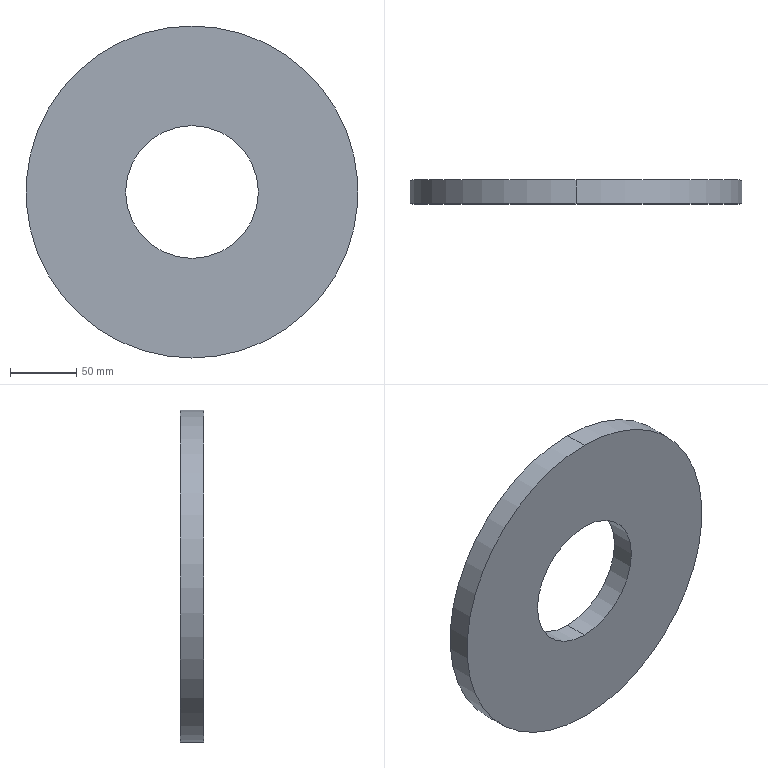Component | SolidWorks | Support4-1 | 1 solid | 6 faces | box 250 x 18 x 250 mm | volume 742201 mm3 | cylinder 4 | plane 2 | commonest cylinder face diameters 100 x2 250 x2 | material Plain Carbon Steel
STEP:
#1=COLOUR_RGB('',0.7922,0.8196,0.9333);
#2=FILL_AREA_STYLE_COLOUR('',#1);
#3=FILL_AREA_STYLE('',(#2));
#4=SURFACE_STYLE_FILL_AREA(#3);
#5=SURFACE_SIDE_STYLE('',(#4));
#6=SURFACE_STYLE_USAGE(.BOTH.,#5);
#7=PRESENTATION_STYLE_ASSIGNMENT((#6));
#8=CARTESIAN_POINT('',(49.235,55.092,74.925));
#9=VERTEX_POINT('',#8);
#10=CARTESIAN_POINT('',(49.235,55.092,70.988));
#11=VERTEX_POINT('',#10);
#12=CARTESIAN_POINT('',(49.235,55.092,72.956));
#13=DIRECTION('',(0.,-1.,-0.));
#14=DIRECTION('',(-0.,0.,-1.));
#15=AXIS2_PLACEMENT_3D('',#12,#13,#14);
#16=CIRCLE('',#15,1.969);
#17=EDGE_CURVE('',#9,#11,#16,.T.);
#18=ORIENTED_EDGE('',*,*,#17,.F.);
#19=CARTESIAN_POINT('',(49.235,54.384,74.925));
#20=VERTEX_POINT('',#19);
#21=CARTESIAN_POINT('',(49.235,55.092,74.925));
#22=DIRECTION('',(0.,-1.,-0.));
#23=VECTOR('',#22,39.37);
#24=LINE('',#21,#23);
#25=EDGE_CURVE('',#9,#20,#24,.T.);
#26=ORIENTED_EDGE('',*,*,#25,.T.);
#27=CARTESIAN_POINT('',(49.235,54.384,70.988));
#28=VERTEX_POINT('',#27);
#29=CARTESIAN_POINT('',(49.235,54.384,72.956));
#30=DIRECTION('',(0.,-1.,-0.));
#31=DIRECTION('',(-0.,0.,-1.));
#32=AXIS2_PLACEMENT_3D('',#29,#30,#31);
#33=CIRCLE('',#32,1.969);
#34=EDGE_CURVE('',#20,#28,#33,.T.);
#35=ORIENTED_EDGE('',*,*,#34,.T.);
#36=CARTESIAN_POINT('',(49.235,55.092,70.988));
#37=DIRECTION('',(0.,-1.,-0.));
#38=VECTOR('',#37,39.37);
#39=LINE('',#36,#38);
#40=EDGE_CURVE('',#11,#28,#39,.T.);
#41=ORIENTED_EDGE('',*,*,#40,.F.);
#42=EDGE_LOOP('',(#18,#26,#35,#41));
#43=FACE_OUTER_BOUND('',#42,.T.);
#44=CARTESIAN_POINT('',(49.235,55.092,72.956));
#45=DIRECTION('',(0.,-1.,-0.));
#46=DIRECTION('',(-0.,0.,-1.));
#47=AXIS2_PLACEMENT_3D('',#44,#45,#46);
#48=CYLINDRICAL_SURFACE('',#47,1.969);
#49=ADVANCED_FACE('',(#43),#48,.F.);
#50=CARTESIAN_POINT('',(49.235,55.092,68.035));
#51=VERTEX_POINT('',#50);
#52=CARTESIAN_POINT('',(49.235,55.092,77.877));
#53=VERTEX_POINT('',#52);
#54=CARTESIAN_POINT('',(49.235,55.092,72.956));
#55=DIRECTION('',(0.,-1.,-0.));
#56=DIRECTION('',(-0.,0.,-1.));
#57=AXIS2_PLACEMENT_3D('',#54,#55,#56);
#58=CIRCLE('',#57,4.921);
#59=EDGE_CURVE('',#51,#53,#58,.T.);
#60=ORIENTED_EDGE('',*,*,#59,.T.);
#61=CARTESIAN_POINT('',(49.235,54.384,77.877));
#62=VERTEX_POINT('',#61);
#63=CARTESIAN_POINT('',(49.235,55.092,77.877));
#64=DIRECTION('',(0.,-1.,-0.));
#65=VECTOR('',#64,39.37);
#66=LINE('',#63,#65);
#67=EDGE_CURVE('',#53,#62,#66,.T.);
#68=ORIENTED_EDGE('',*,*,#67,.T.);
#69=CARTESIAN_POINT('',(49.235,54.384,68.035));
#70=VERTEX_POINT('',#69);
#71=CARTESIAN_POINT('',(49.235,54.384,72.956));
#72=DIRECTION('',(0.,-1.,-0.));
#73=DIRECTION('',(-0.,0.,-1.));
#74=AXIS2_PLACEMENT_3D('',#71,#72,#73);
#75=CIRCLE('',#74,4.921);
#76=EDGE_CURVE('',#70,#62,#75,.T.);
#77=ORIENTED_EDGE('',*,*,#76,.F.);
#78=CARTESIAN_POINT('',(49.235,55.092,68.035));
#79=DIRECTION('',(0.,-1.,-0.));
#80=VECTOR('',#79,39.37);
#81=LINE('',#78,#80);
#82=EDGE_CURVE('',#51,#70,#81,.T.);
#83=ORIENTED_EDGE('',*,*,#82,.F.);
#84=EDGE_LOOP('',(#60,#68,#77,#83));
#85=FACE_OUTER_BOUND('',#84,.T.);
#86=CARTESIAN_POINT('',(49.235,55.092,72.956));
#87=DIRECTION('',(0.,-1.,-0.));
#88=DIRECTION('',(-0.,0.,-1.));
#89=AXIS2_PLACEMENT_3D('',#86,#87,#88);
#90=CYLINDRICAL_SURFACE('',#89,4.921);
#91=ADVANCED_FACE('',(#85),#90,.T.);
#92=ORIENTED_EDGE('',*,*,#67,.F.);
#93=CARTESIAN_POINT('',(49.235,55.092,72.956));
#94=DIRECTION('',(0.,-1.,-0.));
#95=DIRECTION('',(-0.,0.,-1.));
#96=AXIS2_PLACEMENT_3D('',#93,#94,#95);
#97=CIRCLE('',#96,4.921);
#98=EDGE_CURVE('',#53,#51,#97,.T.);
#99=ORIENTED_EDGE('',*,*,#98,.T.);
#100=ORIENTED_EDGE('',*,*,#82,.T.);
#101=CARTESIAN_POINT('',(49.235,54.384,72.956));
#102=DIRECTION('',(0.,-1.,-0.));
#103=DIRECTION('',(-0.,0.,-1.));
#104=AXIS2_PLACEMENT_3D('',#101,#102,#103);
#105=CIRCLE('',#104,4.921);
#106=EDGE_CURVE('',#62,#70,#105,.T.);
#107=ORIENTED_EDGE('',*,*,#106,.F.);
#108=EDGE_LOOP('',(#92,#99,#100,#107));
#109=FACE_OUTER_BOUND('',#108,.T.);
#110=CARTESIAN_POINT('',(49.235,55.092,72.956));
#111=DIRECTION('',(0.,-1.,-0.));
#112=DIRECTION('',(-0.,0.,-1.));
#113=AXIS2_PLACEMENT_3D('',#110,#111,#112);
#114=CYLINDRICAL_SURFACE('',#113,4.921);
#115=ADVANCED_FACE('',(#109),#114,.T.);
#116=CARTESIAN_POINT('',(49.235,55.092,72.956));
#117=DIRECTION('',(0.,-1.,-0.));
#118=DIRECTION('',(-0.,0.,-1.));
#119=AXIS2_PLACEMENT_3D('',#116,#117,#118);
#120=CIRCLE('',#119,1.969);
#121=EDGE_CURVE('',#11,#9,#120,.T.);
#122=ORIENTED_EDGE('',*,*,#121,.T.);
#123=ORIENTED_EDGE('',*,*,#17,.T.);
#124=EDGE_LOOP('',(#122,#123));
#125=FACE_BOUND('',#124,.T.);
#126=ORIENTED_EDGE('',*,*,#59,.F.);
#127=ORIENTED_EDGE('',*,*,#98,.F.);
#128=EDGE_LOOP('',(#126,#127));
#129=FACE_OUTER_BOUND('',#128,.T.);
#130=CARTESIAN_POINT('',(49.235,55.092,72.956));
#131=DIRECTION('',(0.,-1.,-0.));
#132=DIRECTION('',(-0.,0.,-1.));
#133=AXIS2_PLACEMENT_3D('',#130,#131,#132);
#134=PLANE('',#133);
#135=ADVANCED_FACE('',(#125,#129),#134,.F.);
#136=CARTESIAN_POINT('',(49.235,54.384,72.956));
#137=DIRECTION('',(0.,-1.,-0.));
#138=DIRECTION('',(-0.,0.,-1.));
#139=AXIS2_PLACEMENT_3D('',#136,#137,#138);
#140=CIRCLE('',#139,1.969);
#141=EDGE_CURVE('',#28,#20,#140,.T.);
#142=ORIENTED_EDGE('',*,*,#141,.F.);
#143=ORIENTED_EDGE('',*,*,#34,.F.);
#144=EDGE_LOOP('',(#142,#143));
#145=FACE_BOUND('',#144,.T.);
#146=ORIENTED_EDGE('',*,*,#76,.T.);
#147=ORIENTED_EDGE('',*,*,#106,.T.);
#148=EDGE_LOOP('',(#146,#147));
#149=FACE_OUTER_BOUND('',#148,.T.);
#150=CARTESIAN_POINT('',(49.235,54.384,72.956));
#151=DIRECTION('',(0.,-1.,-0.));
#152=DIRECTION('',(-0.,0.,-1.));
#153=AXIS2_PLACEMENT_3D('',#150,#151,#152);
#154=PLANE('',#153);
#155=ADVANCED_FACE('',(#145,#149),#154,.T.);
#156=ORIENTED_EDGE('',*,*,#25,.F.);
#157=ORIENTED_EDGE('',*,*,#121,.F.);
#158=ORIENTED_EDGE('',*,*,#40,.T.);
#159=ORIENTED_EDGE('',*,*,#141,.T.);
#160=EDGE_LOOP('',(#156,#157,#158,#159));
#161=FACE_OUTER_BOUND('',#160,.T.);
#162=CARTESIAN_POINT('',(49.235,55.092,72.956));
#163=DIRECTION('',(0.,-1.,-0.));
#164=DIRECTION('',(-0.,0.,-1.));
#165=AXIS2_PLACEMENT_3D('',#162,#163,#164);
#166=CYLINDRICAL_SURFACE('',#165,1.969);
#167=ADVANCED_FACE('',(#161),#166,.F.);
#168=CLOSED_SHELL('',(#49,#91,#115,#135,#155,#167));
#169=MANIFOLD_SOLID_BREP('',#168);
#170=STYLED_ITEM('',(#7),#169);
#171=PRESENTATION_LAYER_ASSIGNMENT('','',(#170));
#172=CARTESIAN_POINT('',(0.,0.,0.));
#173=DIRECTION('',(0.,0.,1.));
#174=DIRECTION('',(1.,0.,0.));
#175=AXIS2_PLACEMENT_3D('',#172,#173,#174);
#176=(LENGTH_UNIT()NAMED_UNIT(*)SI_UNIT($,.METRE.));
#177=LENGTH_MEASURE_WITH_UNIT(LENGTH_MEASURE(0.0254),#176);
#178=DIMENSIONAL_EXPONENTS(1.,0.,0.,0.,0.,0.,0.);
#179=(CONVERSION_BASED_UNIT('',#177)LENGTH_UNIT()NAMED_UNIT(#178));
#180=UNCERTAINTY_MEASURE_WITH_UNIT(LENGTH_MEASURE(0.00001),#179,'','');
#181=(NAMED_UNIT(*)PLANE_ANGLE_UNIT()SI_UNIT($,.RADIAN.));
#182=(NAMED_UNIT(*)SI_UNIT($,.STERADIAN.)SOLID_ANGLE_UNIT());
#183=(GEOMETRIC_REPRESENTATION_CONTEXT(3)GLOBAL_UNCERTAINTY_ASSIGNED_CONTEXT((#180))GLOBAL_UNIT_ASSIGNED_CONTEXT((#179,#181,#182))REPRESENTATION_CONTEXT('',''));
#184=ADVANCED_BREP_SHAPE_REPRESENTATION('',(#169,#175),#183);
#185=(LENGTH_UNIT()NAMED_UNIT(*)SI_UNIT($,.METRE.));
#186=LENGTH_MEASURE_WITH_UNIT(LENGTH_MEASURE(0.0254),#185);
#187=DIMENSIONAL_EXPONENTS(1.,0.,0.,0.,0.,0.,0.);
#188=(CONVERSION_BASED_UNIT('',#186)LENGTH_UNIT()NAMED_UNIT(#187));
#189=UNCERTAINTY_MEASURE_WITH_UNIT(LENGTH_MEASURE(0.00001),#188,'','');
#190=(NAMED_UNIT(*)PLANE_ANGLE_UNIT()SI_UNIT($,.RADIAN.));
#191=(NAMED_UNIT(*)SI_UNIT($,.STERADIAN.)SOLID_ANGLE_UNIT());
#192=(GEOMETRIC_REPRESENTATION_CONTEXT(3)GLOBAL_UNCERTAINTY_ASSIGNED_CONTEXT((#189))GLOBAL_UNIT_ASSIGNED_CONTEXT((#188,#190,#191))REPRESENTATION_CONTEXT('',''));
#193=MECHANICAL_DESIGN_GEOMETRIC_PRESENTATION_REPRESENTATION('',(#170),#192);